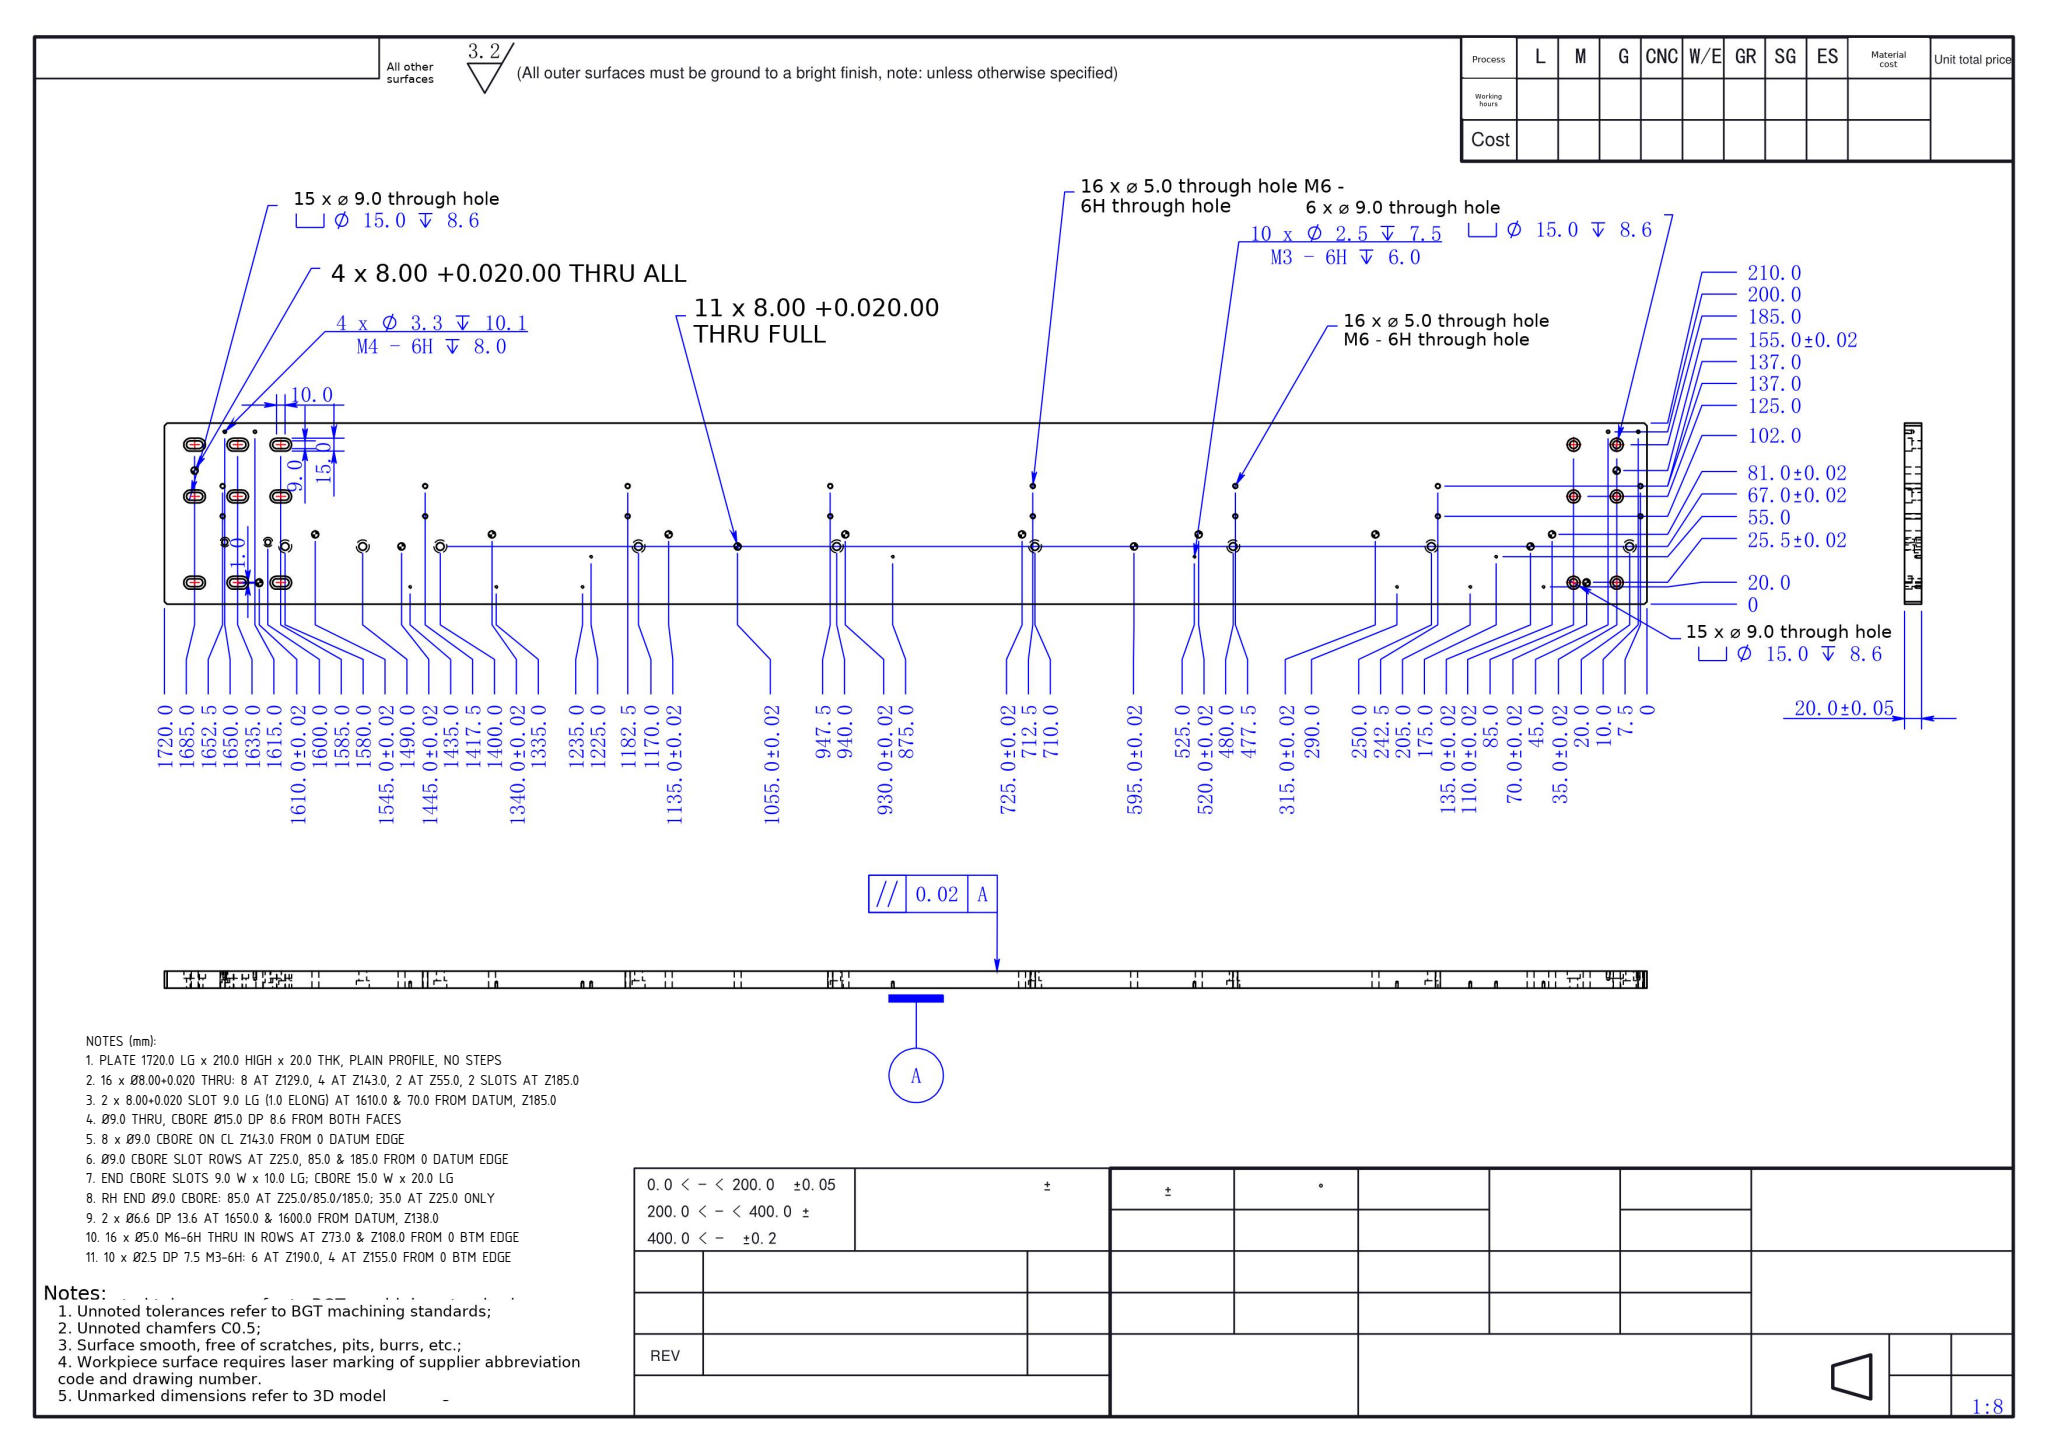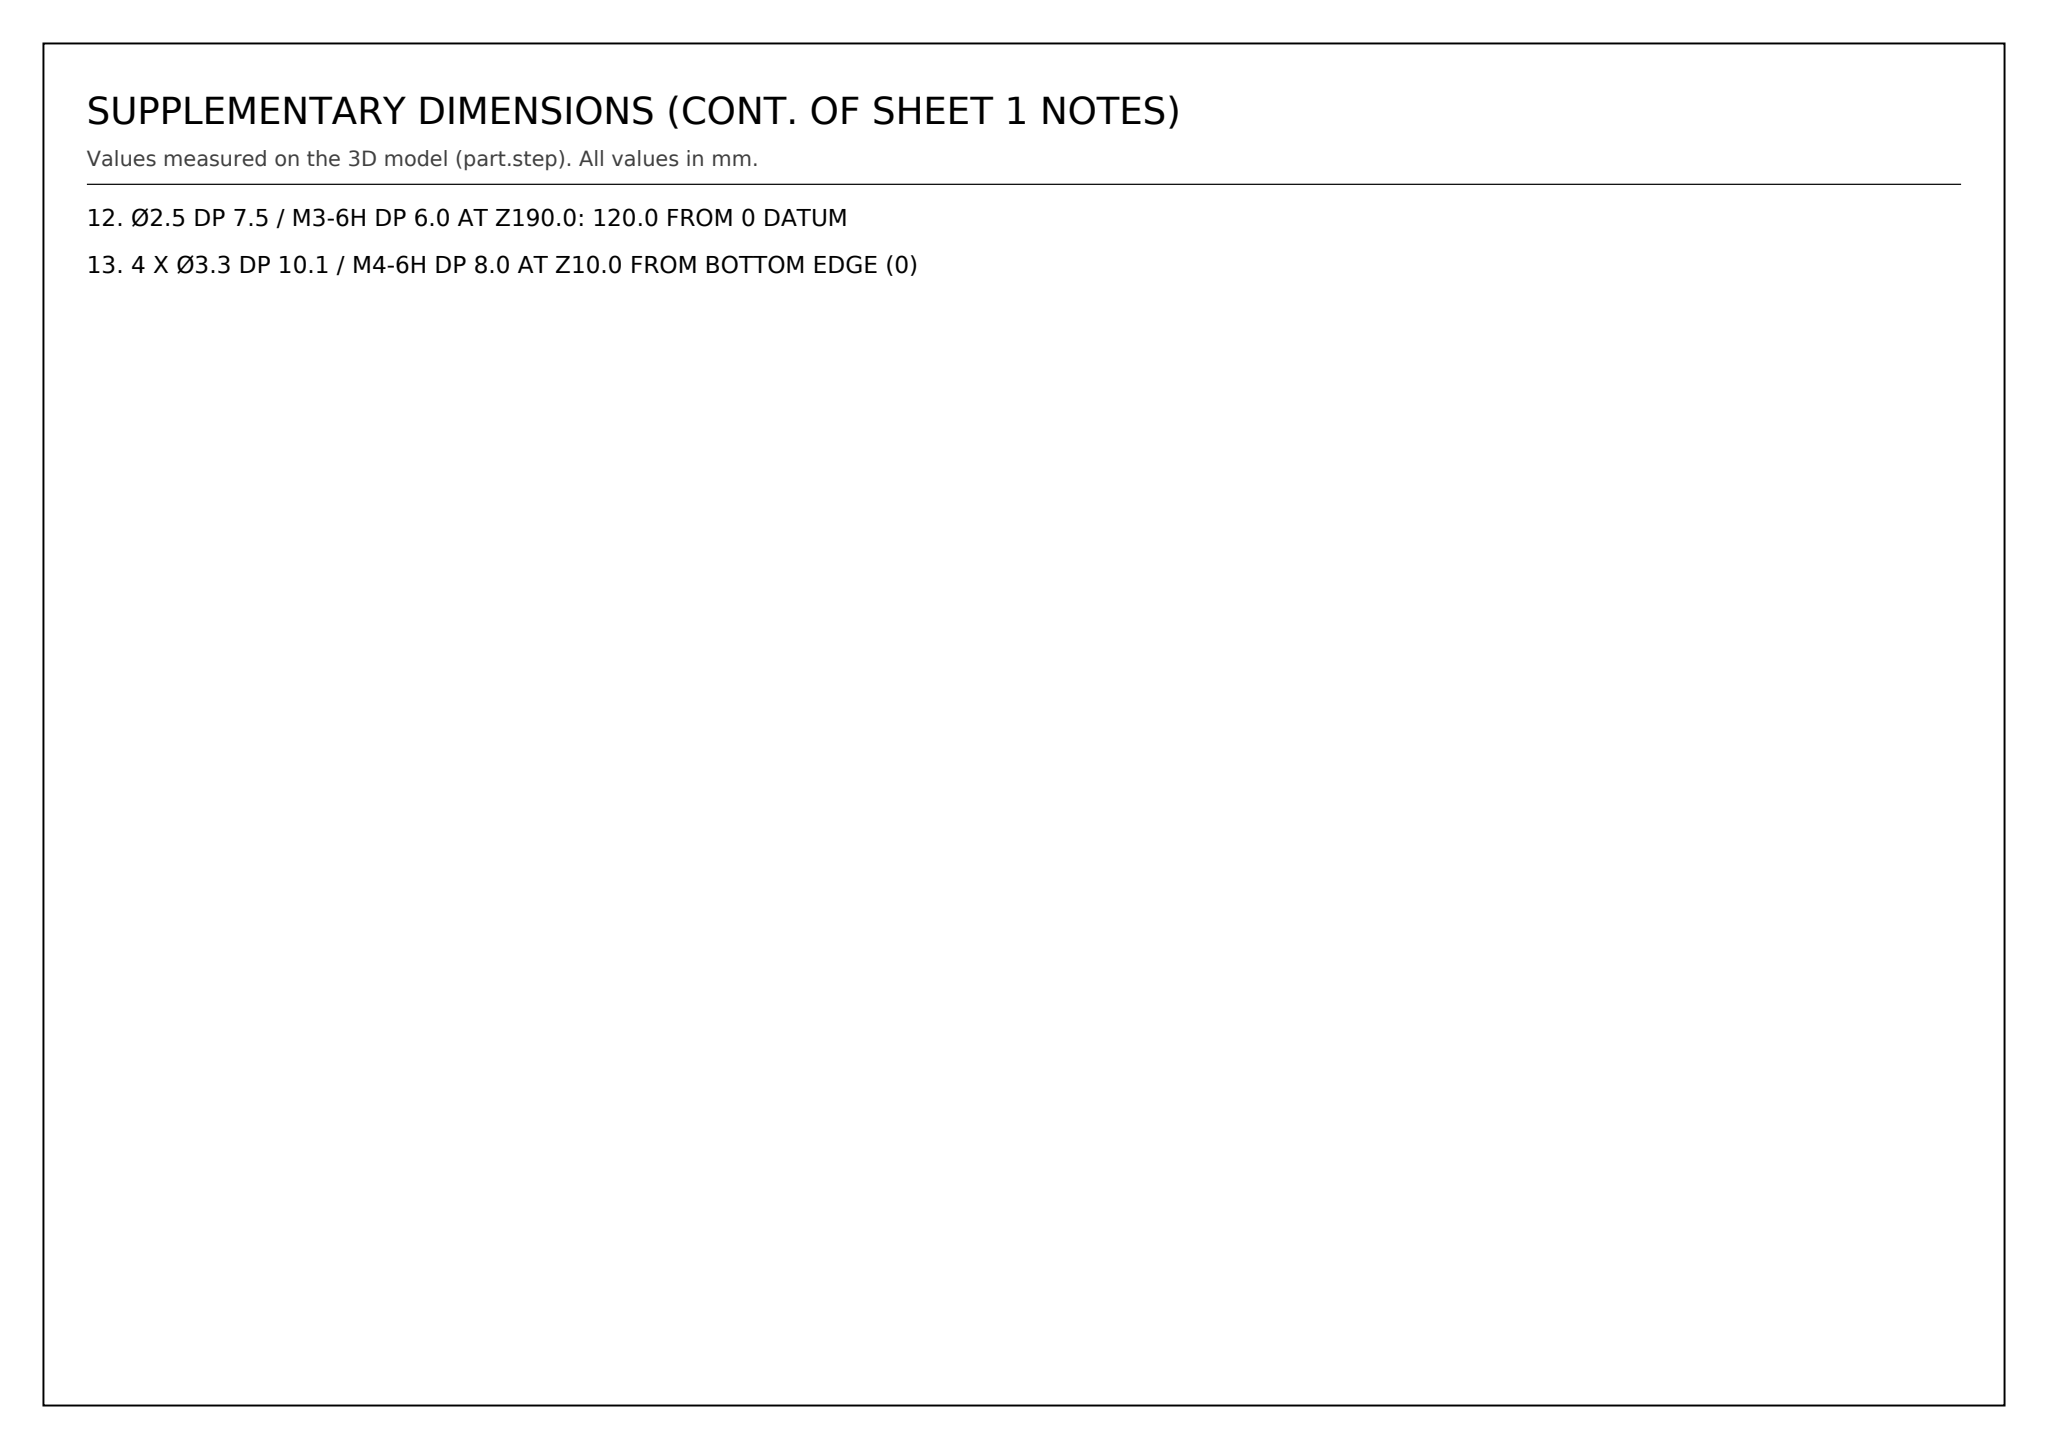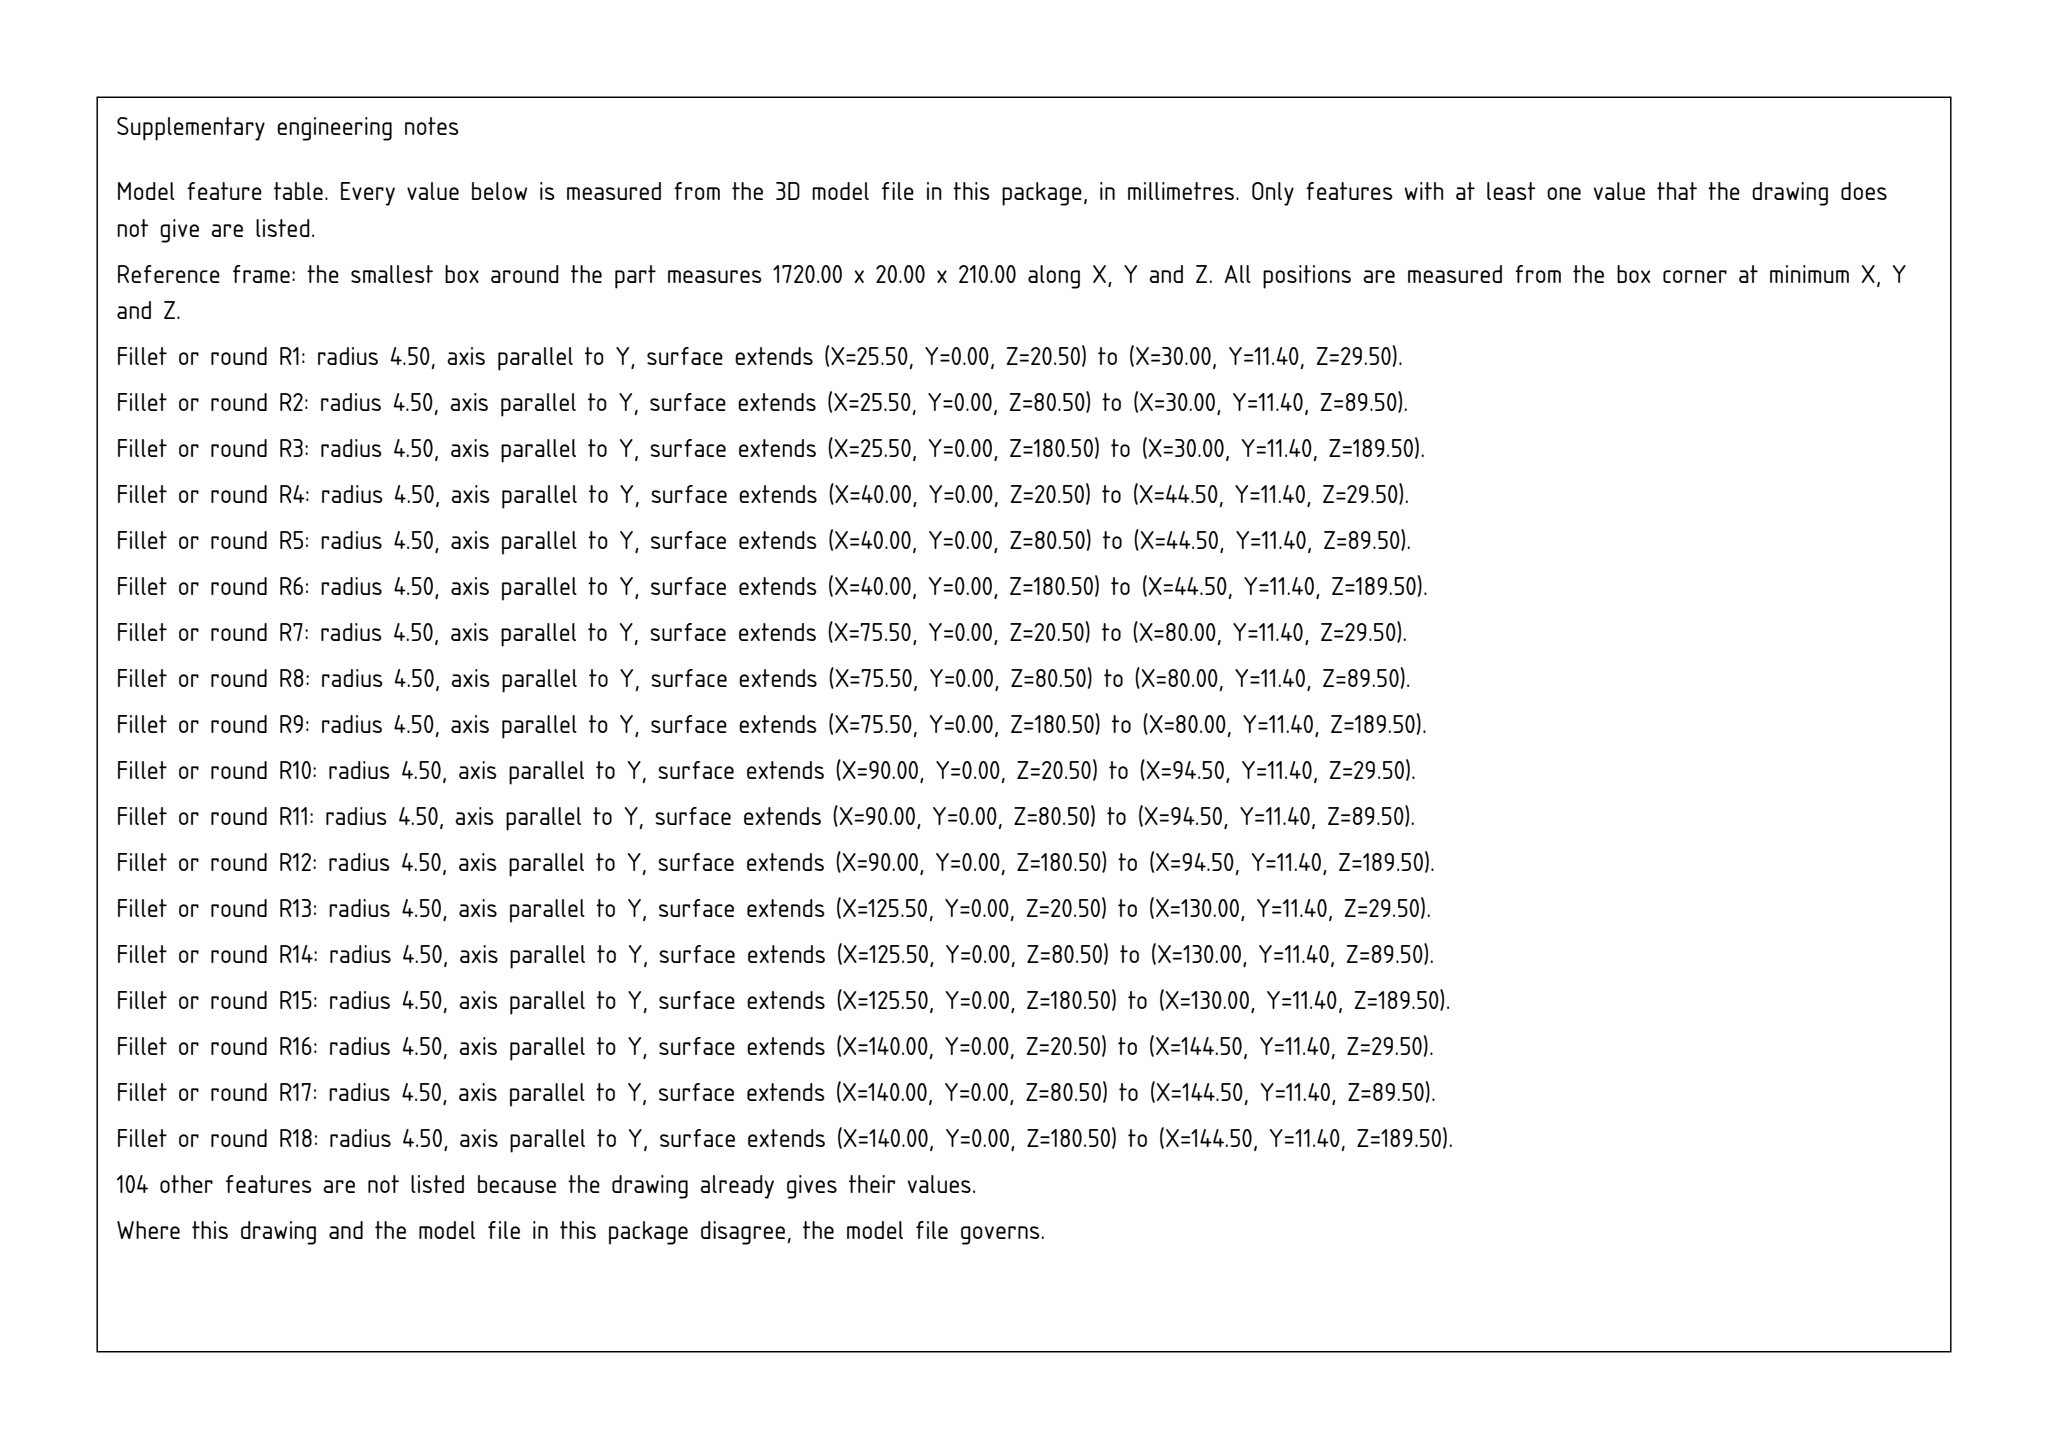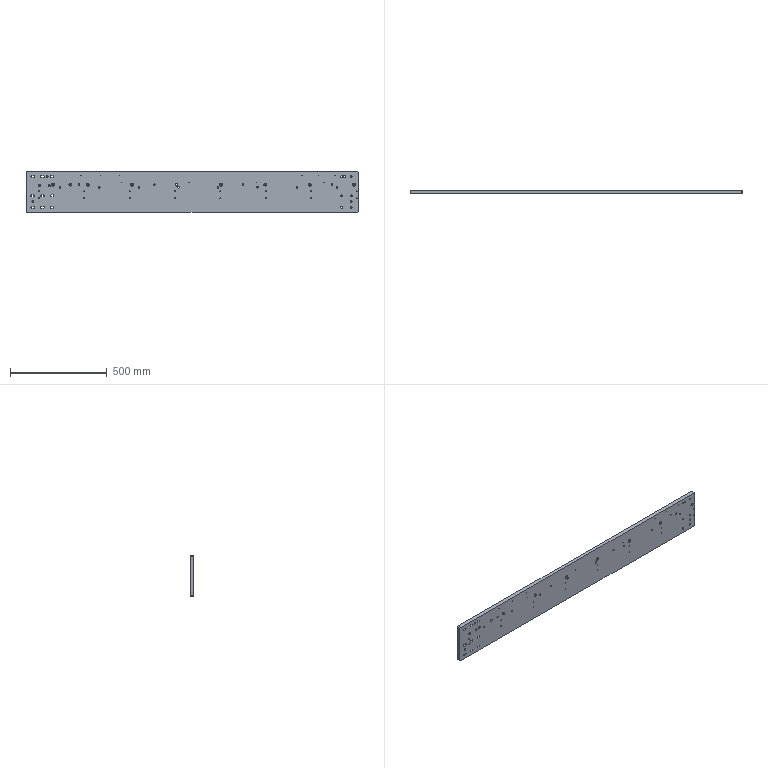Part | SolidWorks | mm | 1 solid | 302 faces | box 1720 x 20 x 210 mm | volume 7123344 mm3 | cylinder 198 | plane 76 | cone 28 | commonest cylinder face diameters 15 x48 9 x48 8 x34 5 x32 2.5 x20 3.3 x8 11 x4 6.6 x4
Drawing notes:
PLATE 1720.0 LG x 210.0 HIGH x 20.0 THK, PLAIN PROFILE, NO STEPS | from the solid: bbox_xyz 1720.0 x 20.0 x 210.0; only faces y=0/20.0 and z=0/210.0
16 x Ø8.00+0.020 THRU: 8 AT Z129.0, 4 AT Z143.0, 2 AT Z55.0, 2 SLOTS AT Z185.0 | from the solid: dia 8.0 L=20 thru: z129 x=175,380,585,790,995,1200,1405,1610; z143 x=275,665,1125,1585; z55 x=35,1685; z185 x=110,1650
2 x 8.00+0.020 SLOT 9.0 LG (1.0 ELONG) AT 1610.0 & 70.0 FROM DATUM, Z185.0 | from the solid: dia 8.0 pairs at x=110 & 1650, z=184.5 and 185.5 (1.0 c/c, 9.0 overall)
Ø9.0 THRU, CBORE Ø15.0 DP 8.6 FROM BOTH FACES | from the solid: y planes 8.6 and 11.4 (=20.0-8.6); dia 9.0 cyls L=11.4 from each face
8 x Ø9.0 CBORE ON CL Z143.0 FROM 0 DATUM EDGE | from the solid: dia 9.0 at z=143.0, x=140,230,320,550,780,1010,1240,1470
Ø9.0 CBORE SLOT ROWS AT Z25.0, 85.0 & 185.0 FROM 0 DATUM EDGE | from the solid: dia 9.0 at z=25/85/185, x=30,40,80,90,130,140,1635,1685
END CBORE SLOTS 9.0 W x 10.0 LG; CBORE 15.0 W x 20.0 LG | from the solid: dia 9.0 pairs x=30&40, 80&90, 130&140; z planes 20.5/29.5 and 17.5/32.5
RH END Ø9.0 CBORE: 85.0 AT Z25.0/85.0/185.0; 35.0 AT Z25.0 ONLY | from the solid: dia 9.0 at x=1635 (85.0 from datum) z=25,85,185; x=1685 (35.0) z=25 only
2 x Ø6.6 DP 13.6 AT 1650.0 & 1600.0 FROM DATUM, Z138.0 | from the solid: dia 6.6 axis y at x=70 & 120, z=138.0, len 13.6
16 x Ø5.0 M6-6H THRU IN ROWS AT Z73.0 & Z108.0 FROM 0 BTM EDGE | from the solid: dia 5.0 cyls L=20 thru, 8 at z=73.0 and 8 at z=108.0
10 x Ø2.5 DP 7.5 M3-6H: 6 AT Z190.0, 4 AT Z155.0 FROM 0 BTM EDGE | from the solid: dia 2.5 L=7.5 at z=190 (x=285,385,485,1430,1515,1600), z=155 (x=495,845,1195,1545)
Ø2.5 DP 7.5 / M3-6H DP 6.0 AT Z190.0: 120.0 FROM 0 DATUM | from the solid: cylinder [2.5,"y",[1600.0,null,190.0],7.5]; bbox X=1720 -> 1720-1600=120 from 0 datum edge
4 X Ø3.3 DP 10.1 / M4-6H DP 8.0 AT Z10.0 FROM BOTTOM EDGE (0) | from the solid: Ø3.3 cyls at z=10.0, x=70,105,1675,1710; depth 10.1, tap M4
build123d program:
from build123d import *

# Parameters (mm, degrees)
SKETCH1_W                                       = 1720
SKETCH1_H                                       = 210
BOSS_EXTRUDE1_DEPTH                             = 20
M8_HEX_SOCKET_HEAD_CAP_SCREW_CBORE1_D           = 9
M8_HEX_SOCKET_HEAD_CAP_SCREW_CBORE1_CBORE_D     = 15
M8_HEX_SOCKET_HEAD_CAP_SCREW_CBORE1_CBORE_DEPTH = 8.6
CHAMFER1_SIZE                                   = 3
M8_HEX_SOCKET_HEAD_CAP_SCREW_CBORE2_D           = 9
M8_HEX_SOCKET_HEAD_CAP_SCREW_CBORE2_CBORE_D     = 15
M8_HEX_SOCKET_HEAD_CAP_SCREW_CBORE2_CBORE_DEPTH = 8.6
M3_TAPPED_HOLE1_D                               = 2.5
M3_TAPPED_HOLE1_DEPTH                           = 7.5
M3_TAPPED_HOLE1_TIP                             = 0.7511
M6_TAPPED_HOLE1_D                               = 5
LPATTERN1_COUNT                                 = 8
LPATTERN1_PITCH                                 = 235
SIZE_MM_DOWEL_PIN_HOLE1_D                       = 8
CUT_EXTRUDE4_DEPTH                              = 1733.888
M4_TAPPED_HOLE1_D                               = 3.3
M4_TAPPED_HOLE1_DEPTH                           = 10.1
M4_TAPPED_HOLE1_TIP                             = 0.9914
CUT_EXTRUDE6_DEPTH                              = 1733.888
CUT_EXTRUDE8_DEPTH                              = 8.6
M6_HEX_SOCKET_HEAD_CAP_SCREW_CBORE1_D           = 6.6
M6_HEX_SOCKET_HEAD_CAP_SCREW_CBORE1_CBORE_D     = 11
M6_HEX_SOCKET_HEAD_CAP_SCREW_CBORE1_CBORE_DEPTH = 6.4
SIZE_MM_DOWEL_PIN_HOLE0_D                       = 8
SIZE_MM_DOWEL_PIN_HOLE4_D                       = 8
LPATTERN3_COUNT                                 = 8
LPATTERN3_PITCH                                 = 205


with BuildPart() as part:
    # Sketch1 → Boss-Extrude1 (new body)
    with BuildSketch(Plane(origin=(0, 0, 0), x_dir=(1, 0, 0), z_dir=(0, 1, 0))):
        with Locations((860, 105)):
            Rectangle(SKETCH1_W, SKETCH1_H)
    extrude(amount=BOSS_EXTRUDE1_DEPTH)

    # M8 Hex Socket Head Cap Screw CBORE1 (through all)
    with Locations(Plane(origin=(0, 20, 0), x_dir=(1, 0, 0), z_dir=(0, 1, 0))):
        with Locations((135, 125), (35, 125), (85, 125), (135, 185), (85, 185), (35, 185), (135, 25), (85, 25), (35, 25), (1635, 25), (1685, 25), (1635, 125), (1685, 125), (1635, 185), (1685, 185)):
            CounterBoreHole(M8_HEX_SOCKET_HEAD_CAP_SCREW_CBORE1_D / 2, M8_HEX_SOCKET_HEAD_CAP_SCREW_CBORE1_CBORE_D / 2, M8_HEX_SOCKET_HEAD_CAP_SCREW_CBORE1_CBORE_DEPTH)

    # Chamfer1
    chamfer1_edges = [part.edges().sort_by_distance(p)[0] for p in [
        (0, 10, -210),
        (1720, 10, -210),
        (1720, 10, 0),
        (0, 10, 0),
    ]]
    chamfer(chamfer1_edges, length=CHAMFER1_SIZE)

    # M8 Hex Socket Head Cap Screw CBORE2 (through all)
    with Locations(Plane(origin=(0, 0, 0), x_dir=(-1, 0, 0), z_dir=(0, -1, 0))):
        with Locations((-1700, 67), (-1470, 67), (-1240, 67), (-1010, 67), (-550, 67), (-320, 67), (-780, 67), (-230, 67), (-140, 67)):
            CounterBoreHole(M8_HEX_SOCKET_HEAD_CAP_SCREW_CBORE2_D / 2, M8_HEX_SOCKET_HEAD_CAP_SCREW_CBORE2_CBORE_D / 2, M8_HEX_SOCKET_HEAD_CAP_SCREW_CBORE2_CBORE_DEPTH)

    # M3 Tapped Hole1
    with Locations(Plane(origin=(0, 0, 0), x_dir=(-1, 0, 0), z_dir=(0, -1, 0))):
        with Locations((-285, 20), (-385, 20), (-485, 20), (-1430, 20), (-1515, 20), (-1600, 20), (-1545, 55), (-1195, 55), (-845, 55), (-495, 55)):
            Hole(M3_TAPPED_HOLE1_D / 2, depth=M3_TAPPED_HOLE1_DEPTH)
            with Locations((0, 0, -(M3_TAPPED_HOLE1_DEPTH + M3_TAPPED_HOLE1_TIP / 2))):  # 118° drill point
                Cone(0, M3_TAPPED_HOLE1_D / 2, M3_TAPPED_HOLE1_TIP, mode=Mode.SUBTRACT)

    # M6 Tapped Hole1 (through all)
    with Locations(Plane(origin=(0, 20, 0), x_dir=(1, 0, 0), z_dir=(0, 1, 0))):
        with Locations((1712.5, 137), (1712.5, 102)):
            m6_tapped_hole1 = Hole(M6_TAPPED_HOLE1_D / 2)

    # LPattern1: M6 Tapped Hole1 ×8
    with Locations(*[(-i * LPATTERN1_PITCH, 0, 0) for i in range(1, LPATTERN1_COUNT)]):
        add(m6_tapped_hole1, mode=Mode.SUBTRACT)

    # Size mm Dowel Pin Hole1 (through all)
    with Locations(Plane(origin=(0, 20, 0), x_dir=(1, 0, 0), z_dir=(0, 1, 0))):
        with Locations((1685, 155), (1650, 25), (35, 155), (110, 25)):
            Hole(SIZE_MM_DOWEL_PIN_HOLE1_D / 2)

    # Sketch20 → Cut-Extrude4 (cut, through all)
    with BuildSketch(Plane(origin=(0, 20, 0), x_dir=(1, 0, 0), z_dir=(0, 1, 0))):
        with BuildLine():
            Line((106, 24.5), (106, 25.5))
            ThreePointArc((106, 25.5), (110, 29.5), (114, 25.5))
            Line((114, 25.5), (114, 24.5))
            ThreePointArc((114, 24.5), (110, 20.5), (106, 24.5))
        make_face()
        with BuildLine():
            Line((1646, 24.5), (1646, 25.5))
            ThreePointArc((1646, 25.5), (1650, 29.5), (1654, 25.5))
            Line((1654, 25.5), (1654, 24.5))
            ThreePointArc((1654, 24.5), (1650, 20.5), (1646, 24.5))
        make_face()
    extrude(amount=-CUT_EXTRUDE4_DEPTH, mode=Mode.SUBTRACT)

    # M4 Tapped Hole1
    with Locations(Plane(origin=(0, 20, 0), x_dir=(1, 0, 0), z_dir=(0, 1, 0))):
        with Locations((1710, 200), (1675, 200), (105, 200), (70, 200)):
            Hole(M4_TAPPED_HOLE1_D / 2, depth=M4_TAPPED_HOLE1_DEPTH)
            with Locations((0, 0, -(M4_TAPPED_HOLE1_DEPTH + M4_TAPPED_HOLE1_TIP / 2))):  # 118° drill point
                Cone(0, M4_TAPPED_HOLE1_D / 2, M4_TAPPED_HOLE1_TIP, mode=Mode.SUBTRACT)

    # Sketch24 → Cut-Extrude6 (cut, through all)
    with BuildSketch(Plane(origin=(0, 20, 0), x_dir=(1, 0, 0), z_dir=(0, 1, 0))):
        with BuildLine():
            Line((30, 189.5), (40, 189.5))
            ThreePointArc((40, 189.5), (44.5, 185), (40, 180.5))
            Line((40, 180.5), (30, 180.5))
            ThreePointArc((30, 180.5), (25.5, 185), (30, 189.5))
        make_face()
        with BuildLine():
            Line((80, 189.5), (90, 189.5))
            ThreePointArc((90, 189.5), (94.5, 185), (90, 180.5))
            Line((90, 180.5), (80, 180.5))
            ThreePointArc((80, 180.5), (75.5, 185), (80, 189.5))
        make_face()
        with BuildLine():
            Line((130, 189.5), (140, 189.5))
            ThreePointArc((140, 189.5), (144.5, 185), (140, 180.5))
            Line((140, 180.5), (130, 180.5))
            ThreePointArc((130, 180.5), (125.5, 185), (130, 189.5))
        make_face()
        with BuildLine():
            Line((30, 129.5), (40, 129.5))
            ThreePointArc((40, 129.5), (44.5, 125), (40, 120.5))
            Line((40, 120.5), (30, 120.5))
            ThreePointArc((30, 120.5), (25.5, 125), (30, 129.5))
        make_face()
        with BuildLine():
            Line((80, 129.5), (90, 129.5))
            ThreePointArc((90, 129.5), (94.5, 125), (90, 120.5))
            Line((90, 120.5), (80, 120.5))
            ThreePointArc((80, 120.5), (75.5, 125), (80, 129.5))
        make_face()
        with BuildLine():
            Line((130, 129.5), (140, 129.5))
            ThreePointArc((140, 129.5), (144.5, 125), (140, 120.5))
            Line((140, 120.5), (130, 120.5))
            ThreePointArc((130, 120.5), (125.5, 125), (130, 129.5))
        make_face()
        with BuildLine():
            Line((30, 29.5), (40, 29.5))
            ThreePointArc((40, 29.5), (44.5, 25), (40, 20.5))
            Line((40, 20.5), (30, 20.5))
            ThreePointArc((30, 20.5), (25.5, 25), (30, 29.5))
        make_face()
        with BuildLine():
            Line((80, 29.5), (90, 29.5))
            ThreePointArc((90, 29.5), (94.5, 25), (90, 20.5))
            Line((90, 20.5), (80, 20.5))
            ThreePointArc((80, 20.5), (75.5, 25), (80, 29.5))
        make_face()
        with BuildLine():
            Line((130, 29.5), (140, 29.5))
            ThreePointArc((140, 29.5), (144.5, 25), (140, 20.5))
            Line((140, 20.5), (130, 20.5))
            ThreePointArc((130, 20.5), (125.5, 25), (130, 29.5))
        make_face()
    extrude(amount=-CUT_EXTRUDE6_DEPTH, mode=Mode.SUBTRACT)

    # Sketch25 → Cut-Extrude8 (cut)
    with BuildSketch(Plane(origin=(0, 20, 0), x_dir=(1, 0, 0), z_dir=(0, 1, 0))):
        with BuildLine():
            Line((30, 192.5), (40, 192.5))
            ThreePointArc((40, 192.5), (47.5, 185), (40, 177.5))
            Line((40, 177.5), (30, 177.5))
            ThreePointArc((30, 177.5), (22.5, 185), (30, 192.5))
        make_face()
        with BuildLine():
            Line((80, 192.5), (90, 192.5))
            ThreePointArc((90, 192.5), (97.5, 185), (90, 177.5))
            Line((90, 177.5), (80, 177.5))
            ThreePointArc((80, 177.5), (72.5, 185), (80, 192.5))
        make_face()
        with BuildLine():
            Line((130, 192.5), (140, 192.5))
            ThreePointArc((140, 192.5), (147.5, 185), (140, 177.5))
            Line((140, 177.5), (130, 177.5))
            ThreePointArc((130, 177.5), (122.5, 185), (130, 192.5))
        make_face()
        with BuildLine():
            Line((30, 132.5), (40, 132.5))
            ThreePointArc((40, 132.5), (47.5, 125), (40, 117.5))
            Line((40, 117.5), (30, 117.5))
            ThreePointArc((30, 117.5), (22.5, 125), (30, 132.5))
        make_face()
        with BuildLine():
            Line((80, 132.5), (90, 132.5))
            ThreePointArc((90, 132.5), (97.5, 125), (90, 117.5))
            Line((90, 117.5), (80, 117.5))
            ThreePointArc((80, 117.5), (72.5, 125), (80, 132.5))
        make_face()
        with BuildLine():
            Line((130, 132.5), (140, 132.5))
            ThreePointArc((140, 132.5), (147.5, 125), (140, 117.5))
            Line((140, 117.5), (130, 117.5))
            ThreePointArc((130, 117.5), (122.5, 125), (130, 132.5))
        make_face()
        with BuildLine():
            Line((30, 32.5), (40, 32.5))
            ThreePointArc((40, 32.5), (47.5, 25), (40, 17.5))
            Line((40, 17.5), (30, 17.5))
            ThreePointArc((30, 17.5), (22.5, 25), (30, 32.5))
        make_face()
        with BuildLine():
            Line((80, 32.5), (90, 32.5))
            ThreePointArc((90, 32.5), (97.5, 25), (90, 17.5))
            Line((90, 17.5), (80, 17.5))
            ThreePointArc((80, 17.5), (72.5, 25), (80, 32.5))
        make_face()
        with BuildLine():
            Line((130, 32.5), (140, 32.5))
            ThreePointArc((140, 32.5), (147.5, 25), (140, 17.5))
            Line((140, 17.5), (130, 17.5))
            ThreePointArc((130, 17.5), (122.5, 25), (130, 32.5))
        make_face()
    extrude(amount=-CUT_EXTRUDE8_DEPTH, mode=Mode.SUBTRACT)

    # M6 Hex Socket Head Cap Screw CBORE1 (through all)
    with Locations(Plane(origin=(0, 0, 0), x_dir=(-1, 0, 0), z_dir=(0, -1, 0))):
        with Locations((-70, 72), (-120, 72)):
            CounterBoreHole(M6_HEX_SOCKET_HEAD_CAP_SCREW_CBORE1_D / 2, M6_HEX_SOCKET_HEAD_CAP_SCREW_CBORE1_CBORE_D / 2, M6_HEX_SOCKET_HEAD_CAP_SCREW_CBORE1_CBORE_DEPTH)

    # Size mm Dowel Pin Hole0 (through all)
    with Locations(Plane(origin=(0, 0, 0), x_dir=(-1, 0, 0), z_dir=(0, -1, 0))):
        with Locations((-275, 67), (-665, 67), (-1125, 67), (-1585, 67)):
            Hole(SIZE_MM_DOWEL_PIN_HOLE0_D / 2)

    # Size mm Dowel Pin Hole4 (through all)
    with Locations(Plane(origin=(0, 20, 0), x_dir=(1, 0, 0), z_dir=(0, 1, 0))):
        with Locations((1610, 81)):
            size_mm_dowel_pin_hole4 = Hole(SIZE_MM_DOWEL_PIN_HOLE4_D / 2)

    # LPattern3: Size mm Dowel Pin Hole4 ×8
    with Locations(*[(-i * LPATTERN3_PITCH, 0, 0) for i in range(1, LPATTERN3_COUNT)]):
        add(size_mm_dowel_pin_hole4, mode=Mode.SUBTRACT)


solid = part.part